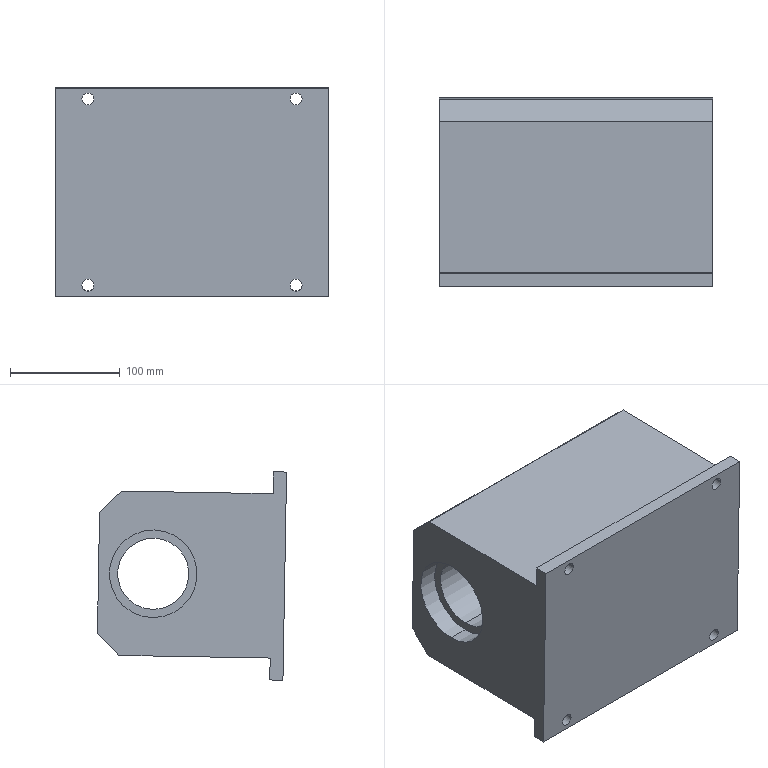Component | SolidWorks | BearingHousing-1 | 1 solid | 28 faces | box 250 x 172.59 x 190.18 mm | volume 5499365 mm3 | cylinder 14 | plane 14 | commonest cylinder face diameters 11 x8 80 x4 65 x2
build123d program:
from build123d import *

# Parameters (mm, degrees)
SKETCH1_W           = 150
SKETCH1_H           = 170
BOSS_EXTRUDE1_DEPTH = 125
SKETCH2_R           = 40
CUT_EXTRUDE1_DEPTH  = 18
SKETCH3_R           = 32.5
CUT_EXTRUDE2_DEPTH  = 259.213
CHAMFER1_SIZE       = 20
SKETCH4_W           = 20
SKETCH4_H           = 250
SKETCH4_R           = 5.5
BOSS_EXTRUDE2_DEPTH = 12


with BuildPart() as part:
    # Sketch1 → Boss-Extrude1 (new, symmetric)
    with BuildSketch(Plane.XY):
        Rectangle(SKETCH1_W, SKETCH1_H)
    extrude(amount=BOSS_EXTRUDE1_DEPTH, both=True)

    # Sketch2 → Cut-Extrude1 (cut)
    with BuildSketch(Plane.XY.offset(125)):
        with Locations((0, 35)):
            Circle(SKETCH2_R)
    cut_extrude1 = extrude(amount=-CUT_EXTRUDE1_DEPTH, mode=Mode.SUBTRACT)

    # Mirror1: Cut-Extrude1 across plane
    add(cut_extrude1.mirror(Plane.XY), mode=Mode.SUBTRACT)

    # Sketch3 → Cut-Extrude2 (cut, through all)
    with BuildSketch(Plane.XY.offset(107)):
        with Locations((0, 35)):
            Circle(SKETCH3_R)
    extrude(amount=-CUT_EXTRUDE2_DEPTH, mode=Mode.SUBTRACT)

    # Chamfer1
    chamfer1_edges = [part.edges().sort_by_distance(p)[0] for p in [
        (-75, 85, 0),
        (75, 85, 0),
    ]]
    chamfer(chamfer1_edges, length=CHAMFER1_SIZE)

    # Sketch4 → Boss-Extrude2 (add)
    # profile 1 of 2: a face of its own
    with BuildSketch(Plane.XZ.offset(85)):
        with Locations((-85, 0)):
            Rectangle(SKETCH4_W, SKETCH4_H)
        with Locations(Location((-85, 95, 0), (0, 0, 270))):
            Circle(SKETCH4_R, mode=Mode.SUBTRACT)
        with Locations(Location((-85, -95, 0), (0, 0, 90))):
            Circle(SKETCH4_R, mode=Mode.SUBTRACT)
    # profile 2 of 2: a face of its own
    with BuildSketch(Plane.XZ.offset(85)):
        with Locations((85, 0)):
            Rectangle(SKETCH4_W, SKETCH4_H)
        with Locations(Location((85, -95, 0), (0, 0, 270))):
            Circle(SKETCH4_R, mode=Mode.SUBTRACT)
        with Locations(Location((85, 95, 0), (0, 0, 90))):
            Circle(SKETCH4_R, mode=Mode.SUBTRACT)
    extrude(amount=-BOSS_EXTRUDE2_DEPTH)


solid = part.part

# Placed as in the assembly
solid = solid.moved(Location((-197.996, 1264.711, 686.505), (1, -90, 0)))
STEP:
#1=COLOUR_RGB('',0.7922,0.8196,0.9333);
#2=FILL_AREA_STYLE_COLOUR('',#1);
#3=FILL_AREA_STYLE('',(#2));
#4=SURFACE_STYLE_FILL_AREA(#3);
#5=SURFACE_SIDE_STYLE('',(#4));
#6=SURFACE_STYLE_USAGE(.BOTH.,#5);
#7=PRESENTATION_STYLE_ASSIGNMENT((#6));
#8=CARTESIAN_POINT('',(-11.752,46.86,30.324));
#9=VERTEX_POINT('',#8);
#10=CARTESIAN_POINT('',(-11.319,46.86,30.324));
#11=VERTEX_POINT('',#10);
#12=CARTESIAN_POINT('',(-11.535,46.86,30.324));
#13=DIRECTION('',(0.,-0.9998,-0.01745));
#14=DIRECTION('',(-1.,0.,0.));
#15=AXIS2_PLACEMENT_3D('',#12,#13,#14);
#16=CIRCLE('',#15,0.2165);
#17=EDGE_CURVE('',#9,#11,#16,.T.);
#18=ORIENTED_EDGE('',*,*,#17,.F.);
#19=CARTESIAN_POINT('',(-11.752,46.387,30.315));
#20=VERTEX_POINT('',#19);
#21=CARTESIAN_POINT('',(-11.752,46.86,30.324));
#22=DIRECTION('',(0.,-0.9998,-0.01745));
#23=VECTOR('',#22,39.37);
#24=LINE('',#21,#23);
#25=EDGE_CURVE('',#9,#20,#24,.T.);
#26=ORIENTED_EDGE('',*,*,#25,.T.);
#27=CARTESIAN_POINT('',(-11.319,46.387,30.315));
#28=VERTEX_POINT('',#27);
#29=CARTESIAN_POINT('',(-11.535,46.387,30.315));
#30=DIRECTION('',(0.,-0.9998,-0.01745));
#31=DIRECTION('',(-1.,0.,0.));
#32=AXIS2_PLACEMENT_3D('',#29,#30,#31);
#33=CIRCLE('',#32,0.2165);
#34=EDGE_CURVE('',#20,#28,#33,.T.);
#35=ORIENTED_EDGE('',*,*,#34,.T.);
#36=CARTESIAN_POINT('',(-11.319,46.86,30.324));
#37=DIRECTION('',(0.,-0.9998,-0.01745));
#38=VECTOR('',#37,39.37);
#39=LINE('',#36,#38);
#40=EDGE_CURVE('',#11,#28,#39,.T.);
#41=ORIENTED_EDGE('',*,*,#40,.F.);
#42=EDGE_LOOP('',(#18,#26,#35,#41));
#43=FACE_OUTER_BOUND('',#42,.T.);
#44=CARTESIAN_POINT('',(-11.535,46.86,30.324));
#45=DIRECTION('',(0.,-0.9998,-0.01745));
#46=DIRECTION('',(1.,0.,0.));
#47=AXIS2_PLACEMENT_3D('',#44,#45,#46);
#48=CYLINDRICAL_SURFACE('',#47,0.2165);
#49=ADVANCED_FACE('',(#43),#48,.F.);
#50=CARTESIAN_POINT('',(-4.271,46.86,30.324));
#51=VERTEX_POINT('',#50);
#52=CARTESIAN_POINT('',(-3.838,46.86,30.324));
#53=VERTEX_POINT('',#52);
#54=CARTESIAN_POINT('',(-4.055,46.86,30.324));
#55=DIRECTION('',(0.,-0.9998,-0.01745));
#56=DIRECTION('',(1.,0.,0.));
#57=AXIS2_PLACEMENT_3D('',#54,#55,#56);
#58=CIRCLE('',#57,0.2165);
#59=EDGE_CURVE('',#51,#53,#58,.T.);
#60=ORIENTED_EDGE('',*,*,#59,.F.);
#61=CARTESIAN_POINT('',(-4.271,46.387,30.315));
#62=VERTEX_POINT('',#61);
#63=CARTESIAN_POINT('',(-4.271,46.86,30.324));
#64=DIRECTION('',(0.,-0.9998,-0.01745));
#65=VECTOR('',#64,39.37);
#66=LINE('',#63,#65);
#67=EDGE_CURVE('',#51,#62,#66,.T.);
#68=ORIENTED_EDGE('',*,*,#67,.T.);
#69=CARTESIAN_POINT('',(-3.838,46.387,30.315));
#70=VERTEX_POINT('',#69);
#71=CARTESIAN_POINT('',(-4.055,46.387,30.315));
#72=DIRECTION('',(0.,-0.9998,-0.01745));
#73=DIRECTION('',(1.,0.,0.));
#74=AXIS2_PLACEMENT_3D('',#71,#72,#73);
#75=CIRCLE('',#74,0.2165);
#76=EDGE_CURVE('',#62,#70,#75,.T.);
#77=ORIENTED_EDGE('',*,*,#76,.T.);
#78=CARTESIAN_POINT('',(-3.838,46.86,30.324));
#79=DIRECTION('',(0.,-0.9998,-0.01745));
#80=VECTOR('',#79,39.37);
#81=LINE('',#78,#80);
#82=EDGE_CURVE('',#53,#70,#81,.T.);
#83=ORIENTED_EDGE('',*,*,#82,.F.);
#84=EDGE_LOOP('',(#60,#68,#77,#83));
#85=FACE_OUTER_BOUND('',#84,.T.);
#86=CARTESIAN_POINT('',(-4.055,46.86,30.324));
#87=DIRECTION('',(0.,-0.9998,-0.01745));
#88=DIRECTION('',(1.,0.,0.));
#89=AXIS2_PLACEMENT_3D('',#86,#87,#88);
#90=CYLINDRICAL_SURFACE('',#89,0.2165);
#91=ADVANCED_FACE('',(#85),#90,.F.);
#92=CARTESIAN_POINT('',(-4.271,46.977,23.632));
#93=VERTEX_POINT('',#92);
#94=CARTESIAN_POINT('',(-3.838,46.977,23.632));
#95=VERTEX_POINT('',#94);
#96=CARTESIAN_POINT('',(-4.055,46.977,23.632));
#97=DIRECTION('',(0.,-0.9998,-0.01745));
#98=DIRECTION('',(-1.,0.,0.));
#99=AXIS2_PLACEMENT_3D('',#96,#97,#98);
#100=CIRCLE('',#99,0.2165);
#101=EDGE_CURVE('',#93,#95,#100,.T.);
#102=ORIENTED_EDGE('',*,*,#101,.F.);
#103=CARTESIAN_POINT('',(-4.271,46.504,23.623));
#104=VERTEX_POINT('',#103);
#105=CARTESIAN_POINT('',(-4.271,46.977,23.632));
#106=DIRECTION('',(0.,-0.9998,-0.01745));
#107=VECTOR('',#106,39.37);
#108=LINE('',#105,#107);
#109=EDGE_CURVE('',#93,#104,#108,.T.);
#110=ORIENTED_EDGE('',*,*,#109,.T.);
#111=CARTESIAN_POINT('',(-3.838,46.504,23.623));
#112=VERTEX_POINT('',#111);
#113=CARTESIAN_POINT('',(-4.055,46.504,23.623));
#114=DIRECTION('',(0.,-0.9998,-0.01745));
#115=DIRECTION('',(-1.,0.,0.));
#116=AXIS2_PLACEMENT_3D('',#113,#114,#115);
#117=CIRCLE('',#116,0.2165);
#118=EDGE_CURVE('',#104,#112,#117,.T.);
#119=ORIENTED_EDGE('',*,*,#118,.T.);
#120=CARTESIAN_POINT('',(-3.838,46.977,23.632));
#121=DIRECTION('',(0.,-0.9998,-0.01745));
#122=VECTOR('',#121,39.37);
#123=LINE('',#120,#122);
#124=EDGE_CURVE('',#95,#112,#123,.T.);
#125=ORIENTED_EDGE('',*,*,#124,.F.);
#126=EDGE_LOOP('',(#102,#110,#119,#125));
#127=FACE_OUTER_BOUND('',#126,.T.);
#128=CARTESIAN_POINT('',(-4.055,46.977,23.632));
#129=DIRECTION('',(0.,-0.9998,-0.01745));
#130=DIRECTION('',(1.,0.,0.));
#131=AXIS2_PLACEMENT_3D('',#128,#129,#130);
#132=CYLINDRICAL_SURFACE('',#131,0.2165);
#133=ADVANCED_FACE('',(#127),#132,.F.);
#134=CARTESIAN_POINT('',(-11.752,46.977,23.632));
#135=VERTEX_POINT('',#134);
#136=CARTESIAN_POINT('',(-11.319,46.977,23.632));
#137=VERTEX_POINT('',#136);
#138=CARTESIAN_POINT('',(-11.535,46.977,23.632));
#139=DIRECTION('',(0.,-0.9998,-0.01745));
#140=DIRECTION('',(1.,0.,0.));
#141=AXIS2_PLACEMENT_3D('',#138,#139,#140);
#142=CIRCLE('',#141,0.2165);
#143=EDGE_CURVE('',#135,#137,#142,.T.);
#144=ORIENTED_EDGE('',*,*,#143,.F.);
#145=CARTESIAN_POINT('',(-11.752,46.504,23.623));
#146=VERTEX_POINT('',#145);
#147=CARTESIAN_POINT('',(-11.752,46.977,23.632));
#148=DIRECTION('',(0.,-0.9998,-0.01745));
#149=VECTOR('',#148,39.37);
#150=LINE('',#147,#149);
#151=EDGE_CURVE('',#135,#146,#150,.T.);
#152=ORIENTED_EDGE('',*,*,#151,.T.);
#153=CARTESIAN_POINT('',(-11.319,46.504,23.623));
#154=VERTEX_POINT('',#153);
#155=CARTESIAN_POINT('',(-11.535,46.504,23.623));
#156=DIRECTION('',(0.,-0.9998,-0.01745));
#157=DIRECTION('',(1.,0.,0.));
#158=AXIS2_PLACEMENT_3D('',#155,#156,#157);
#159=CIRCLE('',#158,0.2165);
#160=EDGE_CURVE('',#146,#154,#159,.T.);
#161=ORIENTED_EDGE('',*,*,#160,.T.);
#162=CARTESIAN_POINT('',(-11.319,46.977,23.632));
#163=DIRECTION('',(0.,-0.9998,-0.01745));
#164=VECTOR('',#163,39.37);
#165=LINE('',#162,#164);
#166=EDGE_CURVE('',#137,#154,#165,.T.);
#167=ORIENTED_EDGE('',*,*,#166,.F.);
#168=EDGE_LOOP('',(#144,#152,#161,#167));
#169=FACE_OUTER_BOUND('',#168,.T.);
#170=CARTESIAN_POINT('',(-11.535,46.977,23.632));
#171=DIRECTION('',(0.,-0.9998,-0.01745));
#172=DIRECTION('',(1.,0.,0.));
#173=AXIS2_PLACEMENT_3D('',#170,#171,#172);
#174=CYLINDRICAL_SURFACE('',#173,0.2165);
#175=ADVANCED_FACE('',(#169),#174,.F.);
#176=CARTESIAN_POINT('',(-3.583,51.147,28.331));
#177=VERTEX_POINT('',#176);
#178=CARTESIAN_POINT('',(-3.583,51.192,25.772));
#179=VERTEX_POINT('',#178);
#180=CARTESIAN_POINT('',(-3.583,51.17,27.052));
#181=DIRECTION('',(1.,0.,0.));
#182=DIRECTION('',(0.,0.01745,-0.9998));
#183=AXIS2_PLACEMENT_3D('',#180,#181,#182);
#184=CIRCLE('',#183,1.28);
#185=EDGE_CURVE('',#177,#179,#184,.T.);
#186=ORIENTED_EDGE('',*,*,#185,.T.);
#187=CARTESIAN_POINT('',(-12.008,51.192,25.772));
#188=VERTEX_POINT('',#187);
#189=CARTESIAN_POINT('',(-2.874,51.192,25.772));
#190=DIRECTION('',(-1.,-0.,-0.));
#191=VECTOR('',#190,39.37);
#192=LINE('',#189,#191);
#193=EDGE_CURVE('',#179,#188,#192,.T.);
#194=ORIENTED_EDGE('',*,*,#193,.T.);
#195=CARTESIAN_POINT('',(-12.008,51.147,28.331));
#196=VERTEX_POINT('',#195);
#197=CARTESIAN_POINT('',(-12.008,51.17,27.052));
#198=DIRECTION('',(-1.,-0.,-0.));
#199=DIRECTION('',(0.,-0.01745,0.9998));
#200=AXIS2_PLACEMENT_3D('',#197,#198,#199);
#201=CIRCLE('',#200,1.28);
#202=EDGE_CURVE('',#188,#196,#201,.T.);
#203=ORIENTED_EDGE('',*,*,#202,.T.);
#204=CARTESIAN_POINT('',(-2.874,51.147,28.331));
#205=DIRECTION('',(-1.,-0.,-0.));
#206=VECTOR('',#205,39.37);
#207=LINE('',#204,#206);
#208=EDGE_CURVE('',#177,#196,#207,.T.);
#209=ORIENTED_EDGE('',*,*,#208,.F.);
#210=EDGE_LOOP('',(#186,#194,#203,#209));
#211=FACE_OUTER_BOUND('',#210,.T.);
#212=CARTESIAN_POINT('',(-2.874,51.17,27.052));
#213=DIRECTION('',(-1.,-0.,-0.));
#214=DIRECTION('',(0.,-0.01745,0.9998));
#215=AXIS2_PLACEMENT_3D('',#212,#213,#214);
#216=CYLINDRICAL_SURFACE('',#215,1.28);
#217=ADVANCED_FACE('',(#211),#216,.F.);
#218=CARTESIAN_POINT('',(-3.583,51.197,25.477));
#219=VERTEX_POINT('',#218);
#220=CARTESIAN_POINT('',(-3.583,51.142,28.626));
#221=VERTEX_POINT('',#220);
#222=CARTESIAN_POINT('',(-3.583,51.17,27.052));
#223=DIRECTION('',(-1.,-0.,-0.));
#224=DIRECTION('',(0.,-0.01745,0.9998));
#225=AXIS2_PLACEMENT_3D('',#222,#223,#224);
#226=CIRCLE('',#225,1.575);
#227=EDGE_CURVE('',#219,#221,#226,.T.);
#228=ORIENTED_EDGE('',*,*,#227,.T.);
#229=CARTESIAN_POINT('',(-2.874,51.142,28.626));
#230=VERTEX_POINT('',#229);
#231=CARTESIAN_POINT('',(-3.583,51.142,28.626));
#232=DIRECTION('',(1.,0.,0.));
#233=VECTOR('',#232,39.37);
#234=LINE('',#231,#233);
#235=EDGE_CURVE('',#221,#230,#234,.T.);
#236=ORIENTED_EDGE('',*,*,#235,.T.);
#237=CARTESIAN_POINT('',(-2.874,51.197,25.477));
#238=VERTEX_POINT('',#237);
#239=CARTESIAN_POINT('',(-2.874,51.17,27.052));
#240=DIRECTION('',(-1.,-0.,-0.));
#241=DIRECTION('',(0.,-0.01745,0.9998));
#242=AXIS2_PLACEMENT_3D('',#239,#240,#241);
#243=CIRCLE('',#242,1.575);
#244=EDGE_CURVE('',#238,#230,#243,.T.);
#245=ORIENTED_EDGE('',*,*,#244,.F.);
#246=CARTESIAN_POINT('',(-3.583,51.197,25.477));
#247=DIRECTION('',(1.,0.,0.));
#248=VECTOR('',#247,39.37);
#249=LINE('',#246,#248);
#250=EDGE_CURVE('',#219,#238,#249,.T.);
#251=ORIENTED_EDGE('',*,*,#250,.F.);
#252=EDGE_LOOP('',(#228,#236,#245,#251));
#253=FACE_OUTER_BOUND('',#252,.T.);
#254=CARTESIAN_POINT('',(-3.583,51.17,27.052));
#255=DIRECTION('',(1.,0.,0.));
#256=DIRECTION('',(0.,0.01745,-0.9998));
#257=AXIS2_PLACEMENT_3D('',#254,#255,#256);
#258=CYLINDRICAL_SURFACE('',#257,1.575);
#259=ADVANCED_FACE('',(#253),#258,.F.);
#260=CARTESIAN_POINT('',(-12.008,51.197,25.477));
#261=VERTEX_POINT('',#260);
#262=CARTESIAN_POINT('',(-12.008,51.142,28.626));
#263=VERTEX_POINT('',#262);
#264=CARTESIAN_POINT('',(-12.008,51.17,27.052));
#265=DIRECTION('',(-1.,-0.,-0.));
#266=DIRECTION('',(0.,-0.01745,0.9998));
#267=AXIS2_PLACEMENT_3D('',#264,#265,#266);
#268=CIRCLE('',#267,1.575);
#269=EDGE_CURVE('',#261,#263,#268,.T.);
#270=ORIENTED_EDGE('',*,*,#269,.F.);
#271=CARTESIAN_POINT('',(-12.716,51.197,25.477));
#272=VERTEX_POINT('',#271);
#273=CARTESIAN_POINT('',(-12.008,51.197,25.477));
#274=DIRECTION('',(-1.,-0.,-0.));
#275=VECTOR('',#274,39.37);
#276=LINE('',#273,#275);
#277=EDGE_CURVE('',#261,#272,#276,.T.);
#278=ORIENTED_EDGE('',*,*,#277,.T.);
#279=CARTESIAN_POINT('',(-12.716,51.142,28.626));
#280=VERTEX_POINT('',#279);
#281=CARTESIAN_POINT('',(-12.716,51.17,27.052));
#282=DIRECTION('',(-1.,-0.,-0.));
#283=DIRECTION('',(0.,-0.01745,0.9998));
#284=AXIS2_PLACEMENT_3D('',#281,#282,#283);
#285=CIRCLE('',#284,1.575);
#286=EDGE_CURVE('',#272,#280,#285,.T.);
#287=ORIENTED_EDGE('',*,*,#286,.T.);
#288=CARTESIAN_POINT('',(-12.008,51.142,28.626));
#289=DIRECTION('',(-1.,-0.,-0.));
#290=VECTOR('',#289,39.37);
#291=LINE('',#288,#290);
#292=EDGE_CURVE('',#263,#280,#291,.T.);
#293=ORIENTED_EDGE('',*,*,#292,.F.);
#294=EDGE_LOOP('',(#270,#278,#287,#293));
#295=FACE_OUTER_BOUND('',#294,.T.);
#296=CARTESIAN_POINT('',(-12.008,51.17,27.052));
#297=DIRECTION('',(-1.,-0.,-0.));
#298=DIRECTION('',(0.,-0.01745,0.9998));
#299=AXIS2_PLACEMENT_3D('',#296,#297,#298);
#300=CYLINDRICAL_SURFACE('',#299,1.575);
#301=ADVANCED_FACE('',(#295),#300,.F.);
#302=CARTESIAN_POINT('',(-12.716,46.867,29.93));
#303=VERTEX_POINT('',#302);
#304=CARTESIAN_POINT('',(-12.716,52.299,30.025));
#305=VERTEX_POINT('',#304);
#306=CARTESIAN_POINT('',(-12.716,53.086,30.038));
#307=DIRECTION('',(-0.,0.9998,0.01745));
#308=VECTOR('',#307,39.37);
#309=LINE('',#306,#308);
#310=EDGE_CURVE('',#303,#305,#309,.T.);
#311=ORIENTED_EDGE('',*,*,#310,.F.);
#312=CARTESIAN_POINT('',(-2.874,46.867,29.93));
#313=VERTEX_POINT('',#312);
#314=CARTESIAN_POINT('',(-12.716,46.867,29.93));
#315=DIRECTION('',(1.,0.,0.));
#316=VECTOR('',#315,39.37);
#317=LINE('',#314,#316);
#318=EDGE_CURVE('',#303,#313,#317,.T.);
#319=ORIENTED_EDGE('',*,*,#318,.T.);
#320=CARTESIAN_POINT('',(-2.874,52.299,30.025));
#321=VERTEX_POINT('',#320);
#322=CARTESIAN_POINT('',(-2.874,53.086,30.038));
#323=DIRECTION('',(-0.,0.9998,0.01745));
#324=VECTOR('',#323,39.37);
#325=LINE('',#322,#324);
#326=EDGE_CURVE('',#313,#321,#325,.T.);
#327=ORIENTED_EDGE('',*,*,#326,.T.);
#328=CARTESIAN_POINT('',(-12.716,52.299,30.025));
#329=DIRECTION('',(-1.,-0.,-0.));
#330=VECTOR('',#329,39.37);
#331=LINE('',#328,#330);
#332=EDGE_CURVE('',#321,#305,#331,.T.);
#333=ORIENTED_EDGE('',*,*,#332,.T.);
#334=EDGE_LOOP('',(#311,#319,#327,#333));
#335=FACE_OUTER_BOUND('',#334,.T.);
#336=CARTESIAN_POINT('',(-12.716,53.086,30.038));
#337=DIRECTION('',(0.,0.01745,-0.9998));
#338=DIRECTION('',(0.,-0.9998,-0.01745));
#339=AXIS2_PLACEMENT_3D('',#336,#337,#338);
#340=PLANE('',#339);
#341=ADVANCED_FACE('',(#335),#340,.F.);
#342=CARTESIAN_POINT('',(-2.874,53.1,29.251));
#343=VERTEX_POINT('',#342);
#344=CARTESIAN_POINT('',(-2.874,53.176,24.921));
#345=VERTEX_POINT('',#344);
#346=CARTESIAN_POINT('',(-2.874,53.189,24.134));
#347=DIRECTION('',(0.,0.01745,-0.9998));
#348=VECTOR('',#347,39.37);
#349=LINE('',#346,#348);
#350=EDGE_CURVE('',#343,#345,#349,.T.);
#351=ORIENTED_EDGE('',*,*,#350,.T.);
#352=CARTESIAN_POINT('',(-12.716,53.176,24.921));
#353=VERTEX_POINT('',#352);
#354=CARTESIAN_POINT('',(-12.716,53.176,24.921));
#355=DIRECTION('',(-1.,-0.,-0.));
#356=VECTOR('',#355,39.37);
#357=LINE('',#354,#356);
#358=EDGE_CURVE('',#345,#353,#357,.T.);
#359=ORIENTED_EDGE('',*,*,#358,.T.);
#360=CARTESIAN_POINT('',(-12.716,53.1,29.251));
#361=VERTEX_POINT('',#360);
#362=CARTESIAN_POINT('',(-12.716,53.189,24.134));
#363=DIRECTION('',(0.,0.01745,-0.9998));
#364=VECTOR('',#363,39.37);
#365=LINE('',#362,#364);
#366=EDGE_CURVE('',#361,#353,#365,.T.);
#367=ORIENTED_EDGE('',*,*,#366,.F.);
#368=CARTESIAN_POINT('',(-12.716,53.1,29.251));
#369=DIRECTION('',(1.,0.,0.));
#370=VECTOR('',#369,39.37);
#371=LINE('',#368,#370);
#372=EDGE_CURVE('',#361,#343,#371,.T.);
#373=ORIENTED_EDGE('',*,*,#372,.T.);
#374=EDGE_LOOP('',(#351,#359,#367,#373));
#375=FACE_OUTER_BOUND('',#374,.T.);
#376=CARTESIAN_POINT('',(-12.716,53.189,24.134));
#377=DIRECTION('',(0.,-0.9998,-0.01745));
#378=DIRECTION('',(1.,0.,0.));
#379=AXIS2_PLACEMENT_3D('',#376,#377,#378);
#380=PLANE('',#379);
#381=ADVANCED_FACE('',(#375),#380,.F.);
#382=CARTESIAN_POINT('',(-2.874,52.402,24.12));
#383=VERTEX_POINT('',#382);
#384=CARTESIAN_POINT('',(-2.874,46.97,24.025));
#385=VERTEX_POINT('',#384);
#386=CARTESIAN_POINT('',(-2.874,53.189,24.134));
#387=DIRECTION('',(0.,-0.9998,-0.01745));
#388=VECTOR('',#387,39.37);
#389=LINE('',#386,#388);
#390=EDGE_CURVE('',#383,#385,#389,.T.);
#391=ORIENTED_EDGE('',*,*,#390,.T.);
#392=CARTESIAN_POINT('',(-12.716,46.97,24.025));
#393=VERTEX_POINT('',#392);
#394=CARTESIAN_POINT('',(-12.716,46.97,24.025));
#395=DIRECTION('',(-1.,-0.,-0.));
#396=VECTOR('',#395,39.37);
#397=LINE('',#394,#396);
#398=EDGE_CURVE('',#385,#393,#397,.T.);
#399=ORIENTED_EDGE('',*,*,#398,.T.);
#400=CARTESIAN_POINT('',(-12.716,52.402,24.12));
#401=VERTEX_POINT('',#400);
#402=CARTESIAN_POINT('',(-12.716,53.189,24.134));
#403=DIRECTION('',(0.,-0.9998,-0.01745));
#404=VECTOR('',#403,39.37);
#405=LINE('',#402,#404);
#406=EDGE_CURVE('',#401,#393,#405,.T.);
#407=ORIENTED_EDGE('',*,*,#406,.F.);
#408=CARTESIAN_POINT('',(-12.716,52.402,24.12));
#409=DIRECTION('',(1.,0.,0.));
#410=VECTOR('',#409,39.37);
#411=LINE('',#408,#410);
#412=EDGE_CURVE('',#401,#383,#411,.T.);
#413=ORIENTED_EDGE('',*,*,#412,.T.);
#414=EDGE_LOOP('',(#391,#399,#407,#413));
#415=FACE_OUTER_BOUND('',#414,.T.);
#416=CARTESIAN_POINT('',(-12.716,53.189,24.134));
#417=DIRECTION('',(-0.,-0.01745,0.9998));
#418=DIRECTION('',(-0.,0.9998,0.01745));
#419=AXIS2_PLACEMENT_3D('',#416,#417,#418);
#420=PLANE('',#419);
#421=ADVANCED_FACE('',(#415),#420,.F.);
#422=CARTESIAN_POINT('',(-2.874,46.511,23.23));
#423=VERTEX_POINT('',#422);
#424=CARTESIAN_POINT('',(-2.874,46.381,30.709));
#425=VERTEX_POINT('',#424);
#426=CARTESIAN_POINT('',(-2.874,46.497,24.017));
#427=DIRECTION('',(-0.,-0.01745,0.9998));
#428=VECTOR('',#427,39.37);
#429=LINE('',#426,#428);
#430=EDGE_CURVE('',#423,#425,#429,.T.);
#431=ORIENTED_EDGE('',*,*,#430,.T.);
#432=CARTESIAN_POINT('',(-12.716,46.381,30.709));
#433=VERTEX_POINT('',#432);
#434=CARTESIAN_POINT('',(-12.716,46.381,30.709));
#435=DIRECTION('',(-1.,-0.,-0.));
#436=VECTOR('',#435,39.37);
#437=LINE('',#434,#436);
#438=EDGE_CURVE('',#425,#433,#437,.T.);
#439=ORIENTED_EDGE('',*,*,#438,.T.);
#440=CARTESIAN_POINT('',(-12.716,46.511,23.23));
#441=VERTEX_POINT('',#440);
#442=CARTESIAN_POINT('',(-12.716,46.497,24.017));
#443=DIRECTION('',(-0.,-0.01745,0.9998));
#444=VECTOR('',#443,39.37);
#445=LINE('',#442,#444);
#446=EDGE_CURVE('',#441,#433,#445,.T.);
#447=ORIENTED_EDGE('',*,*,#446,.F.);
#448=CARTESIAN_POINT('',(-12.716,46.511,23.23));
#449=DIRECTION('',(1.,0.,0.));
#450=VECTOR('',#449,39.37);
#451=LINE('',#448,#450);
#452=EDGE_CURVE('',#441,#423,#451,.T.);
#453=ORIENTED_EDGE('',*,*,#452,.T.);
#454=EDGE_LOOP('',(#431,#439,#447,#453));
#455=FACE_OUTER_BOUND('',#454,.T.);
#456=CARTESIAN_POINT('',(-4.055,46.504,23.623));
#457=DIRECTION('',(0.,-0.9998,-0.01745));
#458=DIRECTION('',(-1.,0.,0.));
#459=AXIS2_PLACEMENT_3D('',#456,#457,#458);
#460=CIRCLE('',#459,0.2165);
#461=EDGE_CURVE('',#112,#104,#460,.T.);
#462=ORIENTED_EDGE('',*,*,#461,.F.);
#463=ORIENTED_EDGE('',*,*,#118,.F.);
#464=EDGE_LOOP('',(#462,#463));
#465=FACE_BOUND('',#464,.T.);
#466=CARTESIAN_POINT('',(-11.535,46.504,23.623));
#467=DIRECTION('',(0.,-0.9998,-0.01745));
#468=DIRECTION('',(1.,0.,0.));
#469=AXIS2_PLACEMENT_3D('',#466,#467,#468);
#470=CIRCLE('',#469,0.2165);
#471=EDGE_CURVE('',#154,#146,#470,.T.);
#472=ORIENTED_EDGE('',*,*,#471,.F.);
#473=ORIENTED_EDGE('',*,*,#160,.F.);
#474=EDGE_LOOP('',(#472,#473));
#475=FACE_BOUND('',#474,.T.);
#476=CARTESIAN_POINT('',(-11.535,46.387,30.315));
#477=DIRECTION('',(0.,-0.9998,-0.01745));
#478=DIRECTION('',(-1.,0.,0.));
#479=AXIS2_PLACEMENT_3D('',#476,#477,#478);
#480=CIRCLE('',#479,0.2165);
#481=EDGE_CURVE('',#28,#20,#480,.T.);
#482=ORIENTED_EDGE('',*,*,#481,.F.);
#483=ORIENTED_EDGE('',*,*,#34,.F.);
#484=EDGE_LOOP('',(#482,#483));
#485=FACE_BOUND('',#484,.T.);
#486=CARTESIAN_POINT('',(-4.055,46.387,30.315));
#487=DIRECTION('',(0.,-0.9998,-0.01745));
#488=DIRECTION('',(1.,0.,0.));
#489=AXIS2_PLACEMENT_3D('',#486,#487,#488);
#490=CIRCLE('',#489,0.2165);
#491=EDGE_CURVE('',#70,#62,#490,.T.);
#492=ORIENTED_EDGE('',*,*,#491,.F.);
#493=ORIENTED_EDGE('',*,*,#76,.F.);
#494=EDGE_LOOP('',(#492,#493));
#495=FACE_BOUND('',#494,.T.);
#496=CARTESIAN_POINT('',(-12.716,46.497,24.017));
#497=DIRECTION('',(-0.,0.9998,0.01745));
#498=DIRECTION('',(-1.,-0.,-0.));
#499=AXIS2_PLACEMENT_3D('',#496,#497,#498);
#500=PLANE('',#499);
#501=ADVANCED_FACE('',(#455,#465,#475,#485,#495),#500,.F.);
#502=CARTESIAN_POINT('',(-12.716,51.17,27.052));
#503=DIRECTION('',(-1.,-0.,-0.));
#504=DIRECTION('',(0.,-0.01745,0.9998));
#505=AXIS2_PLACEMENT_3D('',#502,#503,#504);
#506=CIRCLE('',#505,1.575);
#507=EDGE_CURVE('',#280,#272,#506,.T.);
#508=ORIENTED_EDGE('',*,*,#507,.F.);
#509=ORIENTED_EDGE('',*,*,#286,.F.);
#510=EDGE_LOOP('',(#508,#509));
#511=FACE_BOUND('',#510,.T.);
#512=ORIENTED_EDGE('',*,*,#366,.T.);
#513=CARTESIAN_POINT('',(-12.716,52.595,24.32));
#514=DIRECTION('',(0.,-0.6947,-0.7193));
#515=VECTOR('',#514,39.37);
#516=LINE('',#513,#515);
#517=EDGE_CURVE('',#353,#401,#516,.T.);
#518=ORIENTED_EDGE('',*,*,#517,.T.);
#519=ORIENTED_EDGE('',*,*,#406,.T.);
#520=CARTESIAN_POINT('',(-12.716,46.983,23.238));
#521=VERTEX_POINT('',#520);
#522=CARTESIAN_POINT('',(-12.716,46.97,24.025));
#523=DIRECTION('',(0.,0.01745,-0.9998));
#524=VECTOR('',#523,39.37);
#525=LINE('',#522,#524);
#526=EDGE_CURVE('',#393,#521,#525,.T.);
#527=ORIENTED_EDGE('',*,*,#526,.T.);
#528=CARTESIAN_POINT('',(-12.716,46.983,23.238));
#529=DIRECTION('',(0.,-0.9998,-0.01745));
#530=VECTOR('',#529,39.37);
#531=LINE('',#528,#530);
#532=EDGE_CURVE('',#521,#441,#531,.T.);
#533=ORIENTED_EDGE('',*,*,#532,.T.);
#534=ORIENTED_EDGE('',*,*,#446,.T.);
#535=CARTESIAN_POINT('',(-12.716,46.853,30.717));
#536=VERTEX_POINT('',#535);
#537=CARTESIAN_POINT('',(-12.716,46.853,30.717));
#538=DIRECTION('',(0.,-0.9998,-0.01745));
#539=VECTOR('',#538,39.37);
#540=LINE('',#537,#539);
#541=EDGE_CURVE('',#536,#433,#540,.T.);
#542=ORIENTED_EDGE('',*,*,#541,.F.);
#543=CARTESIAN_POINT('',(-12.716,46.867,29.93));
#544=DIRECTION('',(0.,0.01745,-0.9998));
#545=VECTOR('',#544,39.37);
#546=LINE('',#543,#545);
#547=EDGE_CURVE('',#536,#303,#546,.T.);
#548=ORIENTED_EDGE('',*,*,#547,.T.);
#549=ORIENTED_EDGE('',*,*,#310,.T.);
#550=CARTESIAN_POINT('',(-12.716,52.499,29.831));
#551=DIRECTION('',(-0.,0.7193,-0.6947));
#552=VECTOR('',#551,39.37);
#553=LINE('',#550,#552);
#554=EDGE_CURVE('',#305,#361,#553,.T.);
#555=ORIENTED_EDGE('',*,*,#554,.T.);
#556=EDGE_LOOP('',(#512,#518,#519,#527,#533,#534,#542,#548,#549,#555));
#557=FACE_OUTER_BOUND('',#556,.T.);
#558=CARTESIAN_POINT('',(-12.716,49.792,27.028));
#559=DIRECTION('',(-1.,-0.,-0.));
#560=DIRECTION('',(-0.,-0.01745,0.9998));
#561=AXIS2_PLACEMENT_3D('',#558,#559,#560);
#562=PLANE('',#561);
#563=ADVANCED_FACE('',(#511,#557),#562,.T.);
#564=ORIENTED_EDGE('',*,*,#244,.T.);
#565=CARTESIAN_POINT('',(-2.874,51.17,27.052));
#566=DIRECTION('',(-1.,-0.,-0.));
#567=DIRECTION('',(0.,-0.01745,0.9998));
#568=AXIS2_PLACEMENT_3D('',#565,#566,#567);
#569=CIRCLE('',#568,1.575);
#570=EDGE_CURVE('',#230,#238,#569,.T.);
#571=ORIENTED_EDGE('',*,*,#570,.T.);
#572=EDGE_LOOP('',(#564,#571));
#573=FACE_BOUND('',#572,.T.);
#574=ORIENTED_EDGE('',*,*,#390,.F.);
#575=CARTESIAN_POINT('',(-2.874,52.402,24.12));
#576=DIRECTION('',(-0.,0.6947,0.7193));
#577=VECTOR('',#576,39.37);
#578=LINE('',#575,#577);
#579=EDGE_CURVE('',#383,#345,#578,.T.);
#580=ORIENTED_EDGE('',*,*,#579,.T.);
#581=ORIENTED_EDGE('',*,*,#350,.F.);
#582=CARTESIAN_POINT('',(-2.874,53.1,29.251));
#583=DIRECTION('',(0.,-0.7193,0.6947));
#584=VECTOR('',#583,39.37);
#585=LINE('',#582,#584);
#586=EDGE_CURVE('',#343,#321,#585,.T.);
#587=ORIENTED_EDGE('',*,*,#586,.T.);
#588=ORIENTED_EDGE('',*,*,#326,.F.);
#589=CARTESIAN_POINT('',(-2.874,46.853,30.717));
#590=VERTEX_POINT('',#589);
#591=CARTESIAN_POINT('',(-2.874,46.867,29.93));
#592=DIRECTION('',(-0.,-0.01745,0.9998));
#593=VECTOR('',#592,39.37);
#594=LINE('',#591,#593);
#595=EDGE_CURVE('',#313,#590,#594,.T.);
#596=ORIENTED_EDGE('',*,*,#595,.T.);
#597=CARTESIAN_POINT('',(-2.874,46.853,30.717));
#598=DIRECTION('',(0.,-0.9998,-0.01745));
#599=VECTOR('',#598,39.37);
#600=LINE('',#597,#599);
#601=EDGE_CURVE('',#590,#425,#600,.T.);
#602=ORIENTED_EDGE('',*,*,#601,.T.);
#603=ORIENTED_EDGE('',*,*,#430,.F.);
#604=CARTESIAN_POINT('',(-2.874,46.983,23.238));
#605=VERTEX_POINT('',#604);
#606=CARTESIAN_POINT('',(-2.874,46.983,23.238));
#607=DIRECTION('',(0.,-0.9998,-0.01745));
#608=VECTOR('',#607,39.37);
#609=LINE('',#606,#608);
#610=EDGE_CURVE('',#605,#423,#609,.T.);
#611=ORIENTED_EDGE('',*,*,#610,.F.);
#612=CARTESIAN_POINT('',(-2.874,46.97,24.025));
#613=DIRECTION('',(-0.,-0.01745,0.9998));
#614=VECTOR('',#613,39.37);
#615=LINE('',#612,#614);
#616=EDGE_CURVE('',#605,#385,#615,.T.);
#617=ORIENTED_EDGE('',*,*,#616,.T.);
#618=EDGE_LOOP('',(#574,#580,#581,#587,#588,#596,#602,#603,#611,#617));
#619=FACE_OUTER_BOUND('',#618,.T.);
#620=CARTESIAN_POINT('',(-2.874,49.792,27.028));
#621=DIRECTION('',(-1.,-0.,-0.));
#622=DIRECTION('',(-0.,-0.01745,0.9998));
#623=AXIS2_PLACEMENT_3D('',#620,#621,#622);
#624=PLANE('',#623);
#625=ADVANCED_FACE('',(#573,#619),#624,.F.);
#626=ORIENTED_EDGE('',*,*,#277,.F.);
#627=CARTESIAN_POINT('',(-12.008,51.17,27.052));
#628=DIRECTION('',(-1.,-0.,-0.));
#629=DIRECTION('',(0.,-0.01745,0.9998));
#630=AXIS2_PLACEMENT_3D('',#627,#628,#629);
#631=CIRCLE('',#630,1.575);
#632=EDGE_CURVE('',#263,#261,#631,.T.);
#633=ORIENTED_EDGE('',*,*,#632,.F.);
#634=ORIENTED_EDGE('',*,*,#292,.T.);
#635=ORIENTED_EDGE('',*,*,#507,.T.);
#636=EDGE_LOOP('',(#626,#633,#634,#635));
#637=FACE_OUTER_BOUND('',#636,.T.);
#638=CARTESIAN_POINT('',(-12.008,51.17,27.052));
#639=DIRECTION('',(-1.,-0.,-0.));
#640=DIRECTION('',(0.,-0.01745,0.9998));
#641=AXIS2_PLACEMENT_3D('',#638,#639,#640);
#642=CYLINDRICAL_SURFACE('',#641,1.575);
#643=ADVANCED_FACE('',(#637),#642,.F.);
#644=CARTESIAN_POINT('',(-12.008,51.17,27.052));
#645=DIRECTION('',(-1.,-0.,-0.));
#646=DIRECTION('',(0.,-0.01745,0.9998));
#647=AXIS2_PLACEMENT_3D('',#644,#645,#646);
#648=CIRCLE('',#647,1.28);
#649=EDGE_CURVE('',#196,#188,#648,.T.);
#650=ORIENTED_EDGE('',*,*,#649,.F.);
#651=ORIENTED_EDGE('',*,*,#202,.F.);
#652=EDGE_LOOP('',(#650,#651));
#653=FACE_BOUND('',#652,.T.);
#654=ORIENTED_EDGE('',*,*,#632,.T.);
#655=ORIENTED_EDGE('',*,*,#269,.T.);
#656=EDGE_LOOP('',(#654,#655));
#657=FACE_OUTER_BOUND('',#656,.T.);
#658=CARTESIAN_POINT('',(-12.008,51.17,27.052));
#659=DIRECTION('',(-1.,-0.,-0.));
#660=DIRECTION('',(-0.,-0.01745,0.9998));
#661=AXIS2_PLACEMENT_3D('',#658,#659,#660);
#662=PLANE('',#661);
#663=ADVANCED_FACE('',(#653,#657),#662,.T.);
#664=ORIENTED_EDGE('',*,*,#235,.F.);
#665=CARTESIAN_POINT('',(-3.583,51.17,27.052));
#666=DIRECTION('',(-1.,-0.,-0.));
#667=DIRECTION('',(0.,-0.01745,0.9998));
#668=AXIS2_PLACEMENT_3D('',#665,#666,#667);
#669=CIRCLE('',#668,1.575);
#670=EDGE_CURVE('',#221,#219,#669,.T.);
#671=ORIENTED_EDGE('',*,*,#670,.T.);
#672=ORIENTED_EDGE('',*,*,#250,.T.);
#673=ORIENTED_EDGE('',*,*,#570,.F.);
#674=EDGE_LOOP('',(#664,#671,#672,#673));
#675=FACE_OUTER_BOUND('',#674,.T.);
#676=CARTESIAN_POINT('',(-3.583,51.17,27.052));
#677=DIRECTION('',(1.,0.,0.));
#678=DIRECTION('',(0.,0.01745,-0.9998));
#679=AXIS2_PLACEMENT_3D('',#676,#677,#678);
#680=CYLINDRICAL_SURFACE('',#679,1.575);
#681=ADVANCED_FACE('',(#675),#680,.F.);
#682=ORIENTED_EDGE('',*,*,#185,.F.);
#683=CARTESIAN_POINT('',(-3.583,51.17,27.052));
#684=DIRECTION('',(1.,0.,0.));
#685=DIRECTION('',(0.,0.01745,-0.9998));
#686=AXIS2_PLACEMENT_3D('',#683,#684,#685);
#687=CIRCLE('',#686,1.28);
#688=EDGE_CURVE('',#179,#177,#687,.T.);
#689=ORIENTED_EDGE('',*,*,#688,.F.);
#690=EDGE_LOOP('',(#682,#689));
#691=FACE_BOUND('',#690,.T.);
#692=ORIENTED_EDGE('',*,*,#227,.F.);
#693=ORIENTED_EDGE('',*,*,#670,.F.);
#694=EDGE_LOOP('',(#692,#693));
#695=FACE_OUTER_BOUND('',#694,.T.);
#696=CARTESIAN_POINT('',(-3.583,51.17,27.052));
#697=DIRECTION('',(1.,0.,0.));
#698=DIRECTION('',(-0.,-0.01745,0.9998));
#699=AXIS2_PLACEMENT_3D('',#696,#697,#698);
#700=PLANE('',#699);
#701=ADVANCED_FACE('',(#691,#695),#700,.T.);
#702=ORIENTED_EDGE('',*,*,#193,.F.);
#703=ORIENTED_EDGE('',*,*,#688,.T.);
#704=ORIENTED_EDGE('',*,*,#208,.T.);
#705=ORIENTED_EDGE('',*,*,#649,.T.);
#706=EDGE_LOOP('',(#702,#703,#704,#705));
#707=FACE_OUTER_BOUND('',#706,.T.);
#708=CARTESIAN_POINT('',(-2.874,51.17,27.052));
#709=DIRECTION('',(-1.,-0.,-0.));
#710=DIRECTION('',(0.,-0.01745,0.9998));
#711=AXIS2_PLACEMENT_3D('',#708,#709,#710);
#712=CYLINDRICAL_SURFACE('',#711,1.28);
#713=ADVANCED_FACE('',(#707),#712,.F.);
#714=ORIENTED_EDGE('',*,*,#517,.F.);
#715=ORIENTED_EDGE('',*,*,#358,.F.);
#716=ORIENTED_EDGE('',*,*,#579,.F.);
#717=ORIENTED_EDGE('',*,*,#412,.F.);
#718=EDGE_LOOP('',(#714,#715,#716,#717));
#719=FACE_OUTER_BOUND('',#718,.T.);
#720=CARTESIAN_POINT('',(-12.716,52.402,24.12));
#721=DIRECTION('',(0.,-0.7193,0.6947));
#722=DIRECTION('',(1.,0.,0.));
#723=AXIS2_PLACEMENT_3D('',#720,#721,#722);
#724=PLANE('',#723);
#725=ADVANCED_FACE('',(#719),#724,.F.);
#726=ORIENTED_EDGE('',*,*,#554,.F.);
#727=ORIENTED_EDGE('',*,*,#332,.F.);
#728=ORIENTED_EDGE('',*,*,#586,.F.);
#729=ORIENTED_EDGE('',*,*,#372,.F.);
#730=EDGE_LOOP('',(#726,#727,#728,#729));
#731=FACE_OUTER_BOUND('',#730,.T.);
#732=CARTESIAN_POINT('',(-12.716,53.1,29.251));
#733=DIRECTION('',(0.,-0.6947,-0.7193));
#734=DIRECTION('',(1.,0.,0.));
#735=AXIS2_PLACEMENT_3D('',#732,#733,#734);
#736=PLANE('',#735);
#737=ADVANCED_FACE('',(#731),#736,.F.);
#738=ORIENTED_EDGE('',*,*,#452,.F.);
#739=ORIENTED_EDGE('',*,*,#532,.F.);
#740=CARTESIAN_POINT('',(-12.716,46.983,23.238));
#741=DIRECTION('',(1.,0.,0.));
#742=VECTOR('',#741,39.37);
#743=LINE('',#740,#742);
#744=EDGE_CURVE('',#521,#605,#743,.T.);
#745=ORIENTED_EDGE('',*,*,#744,.T.);
#746=ORIENTED_EDGE('',*,*,#610,.T.);
#747=EDGE_LOOP('',(#738,#739,#745,#746));
#748=FACE_OUTER_BOUND('',#747,.T.);
#749=CARTESIAN_POINT('',(-12.716,46.983,23.238));
#750=DIRECTION('',(0.,0.01745,-0.9998));
#751=DIRECTION('',(-1.,-0.,-0.));
#752=AXIS2_PLACEMENT_3D('',#749,#750,#751);
#753=PLANE('',#752);
#754=ADVANCED_FACE('',(#748),#753,.T.);
#755=CARTESIAN_POINT('',(-4.055,46.977,23.632));
#756=DIRECTION('',(0.,-0.9998,-0.01745));
#757=DIRECTION('',(-1.,0.,0.));
#758=AXIS2_PLACEMENT_3D('',#755,#756,#757);
#759=CIRCLE('',#758,0.2165);
#760=EDGE_CURVE('',#95,#93,#759,.T.);
#761=ORIENTED_EDGE('',*,*,#760,.T.);
#762=ORIENTED_EDGE('',*,*,#101,.T.);
#763=EDGE_LOOP('',(#761,#762));
#764=FACE_BOUND('',#763,.T.);
#765=CARTESIAN_POINT('',(-11.535,46.977,23.632));
#766=DIRECTION('',(0.,-0.9998,-0.01745));
#767=DIRECTION('',(1.,0.,0.));
#768=AXIS2_PLACEMENT_3D('',#765,#766,#767);
#769=CIRCLE('',#768,0.2165);
#770=EDGE_CURVE('',#137,#135,#769,.T.);
#771=ORIENTED_EDGE('',*,*,#770,.T.);
#772=ORIENTED_EDGE('',*,*,#143,.T.);
#773=EDGE_LOOP('',(#771,#772));
#774=FACE_BOUND('',#773,.T.);
#775=ORIENTED_EDGE('',*,*,#398,.F.);
#776=ORIENTED_EDGE('',*,*,#616,.F.);
#777=ORIENTED_EDGE('',*,*,#744,.F.);
#778=ORIENTED_EDGE('',*,*,#526,.F.);
#779=EDGE_LOOP('',(#775,#776,#777,#778));
#780=FACE_OUTER_BOUND('',#779,.T.);
#781=CARTESIAN_POINT('',(-7.795,46.918,26.978));
#782=DIRECTION('',(-0.,0.9998,0.01745));
#783=DIRECTION('',(-1.,-0.,-0.));
#784=AXIS2_PLACEMENT_3D('',#781,#782,#783);
#785=PLANE('',#784);
#786=ADVANCED_FACE('',(#764,#774,#780),#785,.T.);
#787=ORIENTED_EDGE('',*,*,#151,.F.);
#788=ORIENTED_EDGE('',*,*,#770,.F.);
#789=ORIENTED_EDGE('',*,*,#166,.T.);
#790=ORIENTED_EDGE('',*,*,#471,.T.);
#791=EDGE_LOOP('',(#787,#788,#789,#790));
#792=FACE_OUTER_BOUND('',#791,.T.);
#793=CARTESIAN_POINT('',(-11.535,46.977,23.632));
#794=DIRECTION('',(0.,-0.9998,-0.01745));
#795=DIRECTION('',(1.,0.,0.));
#796=AXIS2_PLACEMENT_3D('',#793,#794,#795);
#797=CYLINDRICAL_SURFACE('',#796,0.2165);
#798=ADVANCED_FACE('',(#792),#797,.F.);
#799=ORIENTED_EDGE('',*,*,#109,.F.);
#800=ORIENTED_EDGE('',*,*,#760,.F.);
#801=ORIENTED_EDGE('',*,*,#124,.T.);
#802=ORIENTED_EDGE('',*,*,#461,.T.);
#803=EDGE_LOOP('',(#799,#800,#801,#802));
#804=FACE_OUTER_BOUND('',#803,.T.);
#805=CARTESIAN_POINT('',(-4.055,46.977,23.632));
#806=DIRECTION('',(0.,-0.9998,-0.01745));
#807=DIRECTION('',(1.,0.,0.));
#808=AXIS2_PLACEMENT_3D('',#805,#806,#807);
#809=CYLINDRICAL_SURFACE('',#808,0.2165);
#810=ADVANCED_FACE('',(#804),#809,.F.);
#811=ORIENTED_EDGE('',*,*,#438,.F.);
#812=ORIENTED_EDGE('',*,*,#601,.F.);
#813=CARTESIAN_POINT('',(-12.716,46.853,30.717));
#814=DIRECTION('',(-1.,-0.,-0.));
#815=VECTOR('',#814,39.37);
#816=LINE('',#813,#815);
#817=EDGE_CURVE('',#590,#536,#816,.T.);
#818=ORIENTED_EDGE('',*,*,#817,.T.);
#819=ORIENTED_EDGE('',*,*,#541,.T.);
#820=EDGE_LOOP('',(#811,#812,#818,#819));
#821=FACE_OUTER_BOUND('',#820,.T.);
#822=CARTESIAN_POINT('',(-12.716,46.853,30.717));
#823=DIRECTION('',(-0.,-0.01745,0.9998));
#824=DIRECTION('',(1.,0.,0.));
#825=AXIS2_PLACEMENT_3D('',#822,#823,#824);
#826=PLANE('',#825);
#827=ADVANCED_FACE('',(#821),#826,.T.);
#828=CARTESIAN_POINT('',(-11.535,46.86,30.324));
#829=DIRECTION('',(0.,-0.9998,-0.01745));
#830=DIRECTION('',(-1.,0.,0.));
#831=AXIS2_PLACEMENT_3D('',#828,#829,#830);
#832=CIRCLE('',#831,0.2165);
#833=EDGE_CURVE('',#11,#9,#832,.T.);
#834=ORIENTED_EDGE('',*,*,#833,.T.);
#835=ORIENTED_EDGE('',*,*,#17,.T.);
#836=EDGE_LOOP('',(#834,#835));
#837=FACE_BOUND('',#836,.T.);
#838=CARTESIAN_POINT('',(-4.055,46.86,30.324));
#839=DIRECTION('',(0.,-0.9998,-0.01745));
#840=DIRECTION('',(1.,0.,0.));
#841=AXIS2_PLACEMENT_3D('',#838,#839,#840);
#842=CIRCLE('',#841,0.2165);
#843=EDGE_CURVE('',#53,#51,#842,.T.);
#844=ORIENTED_EDGE('',*,*,#843,.T.);
#845=ORIENTED_EDGE('',*,*,#59,.T.);
#846=EDGE_LOOP('',(#844,#845));
#847=FACE_BOUND('',#846,.T.);
#848=ORIENTED_EDGE('',*,*,#547,.F.);
#849=ORIENTED_EDGE('',*,*,#817,.F.);
#850=ORIENTED_EDGE('',*,*,#595,.F.);
#851=ORIENTED_EDGE('',*,*,#318,.F.);
#852=EDGE_LOOP('',(#848,#849,#850,#851));
#853=FACE_OUTER_BOUND('',#852,.T.);
#854=CARTESIAN_POINT('',(-7.795,46.918,26.978));
#855=DIRECTION('',(-0.,0.9998,0.01745));
#856=DIRECTION('',(-1.,-0.,-0.));
#857=AXIS2_PLACEMENT_3D('',#854,#855,#856);
#858=PLANE('',#857);
#859=ADVANCED_FACE('',(#837,#847,#853),#858,.T.);
#860=ORIENTED_EDGE('',*,*,#67,.F.);
#861=ORIENTED_EDGE('',*,*,#843,.F.);
#862=ORIENTED_EDGE('',*,*,#82,.T.);
#863=ORIENTED_EDGE('',*,*,#491,.T.);
#864=EDGE_LOOP('',(#860,#861,#862,#863));
#865=FACE_OUTER_BOUND('',#864,.T.);
#866=CARTESIAN_POINT('',(-4.055,46.86,30.324));
#867=DIRECTION('',(0.,-0.9998,-0.01745));
#868=DIRECTION('',(1.,0.,0.));
#869=AXIS2_PLACEMENT_3D('',#866,#867,#868);
#870=CYLINDRICAL_SURFACE('',#869,0.2165);
#871=ADVANCED_FACE('',(#865),#870,.F.);
#872=ORIENTED_EDGE('',*,*,#25,.F.);
#873=ORIENTED_EDGE('',*,*,#833,.F.);
#874=ORIENTED_EDGE('',*,*,#40,.T.);
#875=ORIENTED_EDGE('',*,*,#481,.T.);
#876=EDGE_LOOP('',(#872,#873,#874,#875));
#877=FACE_OUTER_BOUND('',#876,.T.);
#878=CARTESIAN_POINT('',(-11.535,46.86,30.324));
#879=DIRECTION('',(0.,-0.9998,-0.01745));
#880=DIRECTION('',(1.,0.,0.));
#881=AXIS2_PLACEMENT_3D('',#878,#879,#880);
#882=CYLINDRICAL_SURFACE('',#881,0.2165);
#883=ADVANCED_FACE('',(#877),#882,.F.);
#884=CLOSED_SHELL('',(#49,#91,#133,#175,#217,#259,#301,#341,#381,#421,#501,#563,#625,#643,#663,#681,#701,#713,#725,#737,#754,#786,#798,#810,#827,#859,#871,#883));
#885=MANIFOLD_SOLID_BREP('',#884);
#886=STYLED_ITEM('',(#7),#885);
#887=PRESENTATION_LAYER_ASSIGNMENT('','',(#886));
#888=(LENGTH_UNIT()NAMED_UNIT(*)SI_UNIT($,.METRE.));
#889=LENGTH_MEASURE_WITH_UNIT(LENGTH_MEASURE(0.0254),#888);
#890=DIMENSIONAL_EXPONENTS(1.,0.,0.,0.,0.,0.,0.);
#891=(CONVERSION_BASED_UNIT('',#889)LENGTH_UNIT()NAMED_UNIT(#890));
#892=UNCERTAINTY_MEASURE_WITH_UNIT(LENGTH_MEASURE(0.00001),#891,'','');
#893=(NAMED_UNIT(*)PLANE_ANGLE_UNIT()SI_UNIT($,.RADIAN.));
#894=(NAMED_UNIT(*)SI_UNIT($,.STERADIAN.)SOLID_ANGLE_UNIT());
#895=(GEOMETRIC_REPRESENTATION_CONTEXT(3)GLOBAL_UNCERTAINTY_ASSIGNED_CONTEXT((#892))GLOBAL_UNIT_ASSIGNED_CONTEXT((#891,#893,#894))REPRESENTATION_CONTEXT('',''));
#896=MECHANICAL_DESIGN_GEOMETRIC_PRESENTATION_REPRESENTATION('',(#886),#895);
#897=CARTESIAN_POINT('',(0.,0.,0.));
#898=DIRECTION('',(0.,0.,1.));
#899=DIRECTION('',(1.,0.,0.));
#900=AXIS2_PLACEMENT_3D('',#897,#898,#899);
#901=(LENGTH_UNIT()NAMED_UNIT(*)SI_UNIT($,.METRE.));
#902=LENGTH_MEASURE_WITH_UNIT(LENGTH_MEASURE(0.0254),#901);
#903=DIMENSIONAL_EXPONENTS(1.,0.,0.,0.,0.,0.,0.);
#904=(CONVERSION_BASED_UNIT('',#902)LENGTH_UNIT()NAMED_UNIT(#903));
#905=UNCERTAINTY_MEASURE_WITH_UNIT(LENGTH_MEASURE(0.00001),#904,'','');
#906=(NAMED_UNIT(*)PLANE_ANGLE_UNIT()SI_UNIT($,.RADIAN.));
#907=(NAMED_UNIT(*)SI_UNIT($,.STERADIAN.)SOLID_ANGLE_UNIT());
#908=(GEOMETRIC_REPRESENTATION_CONTEXT(3)GLOBAL_UNCERTAINTY_ASSIGNED_CONTEXT((#905))GLOBAL_UNIT_ASSIGNED_CONTEXT((#904,#906,#907))REPRESENTATION_CONTEXT('',''));
#909=ADVANCED_BREP_SHAPE_REPRESENTATION('',(#885,#900),#908);